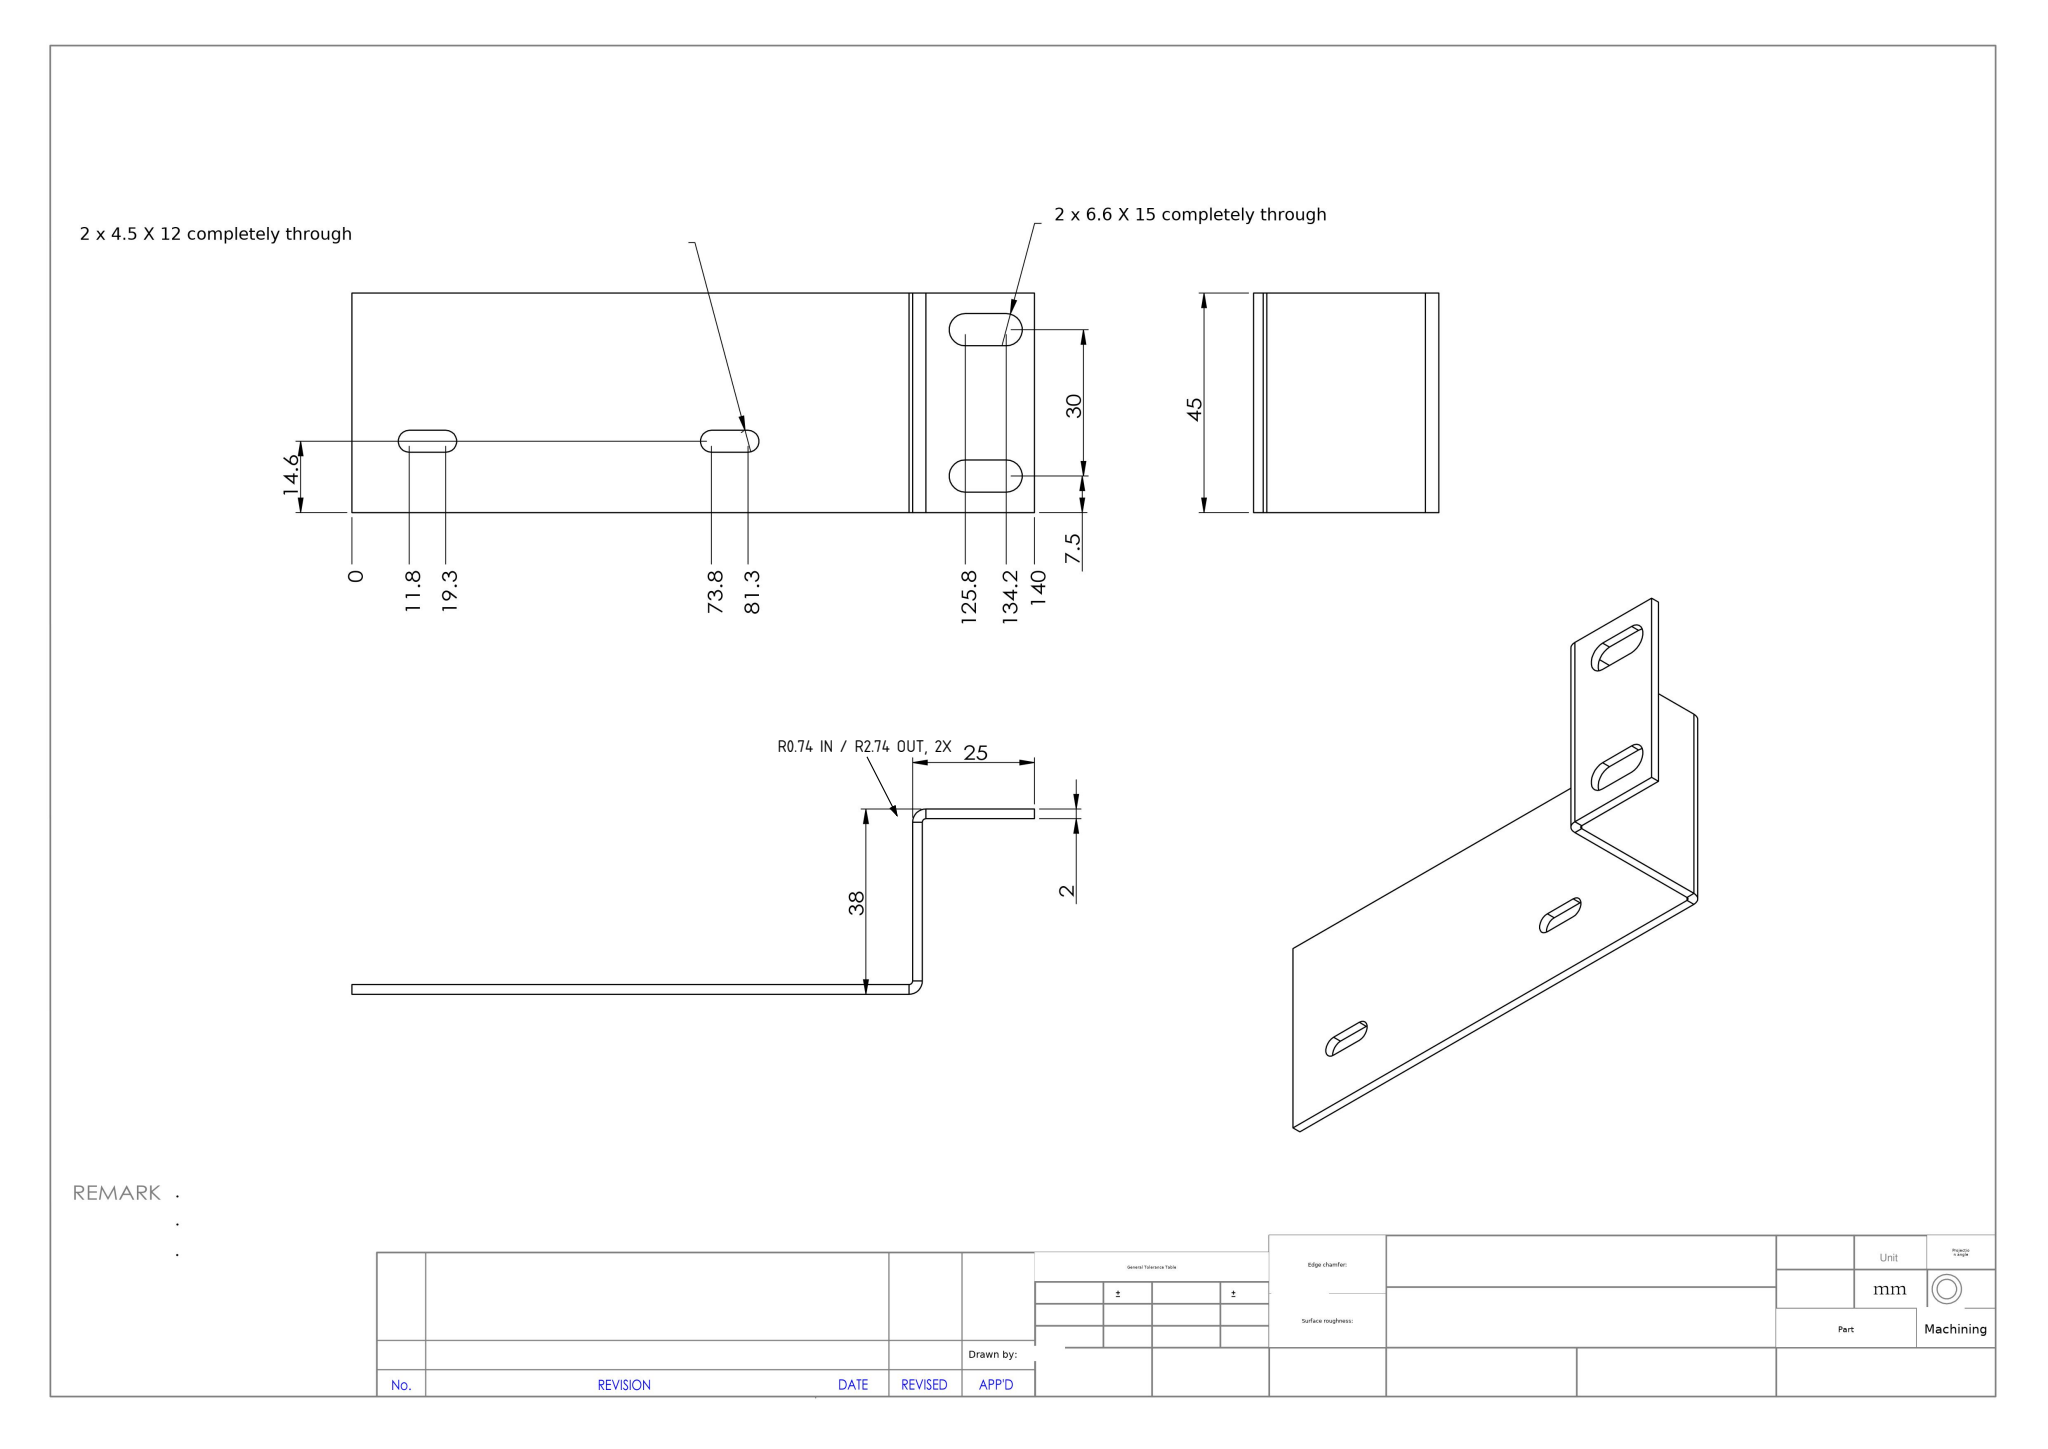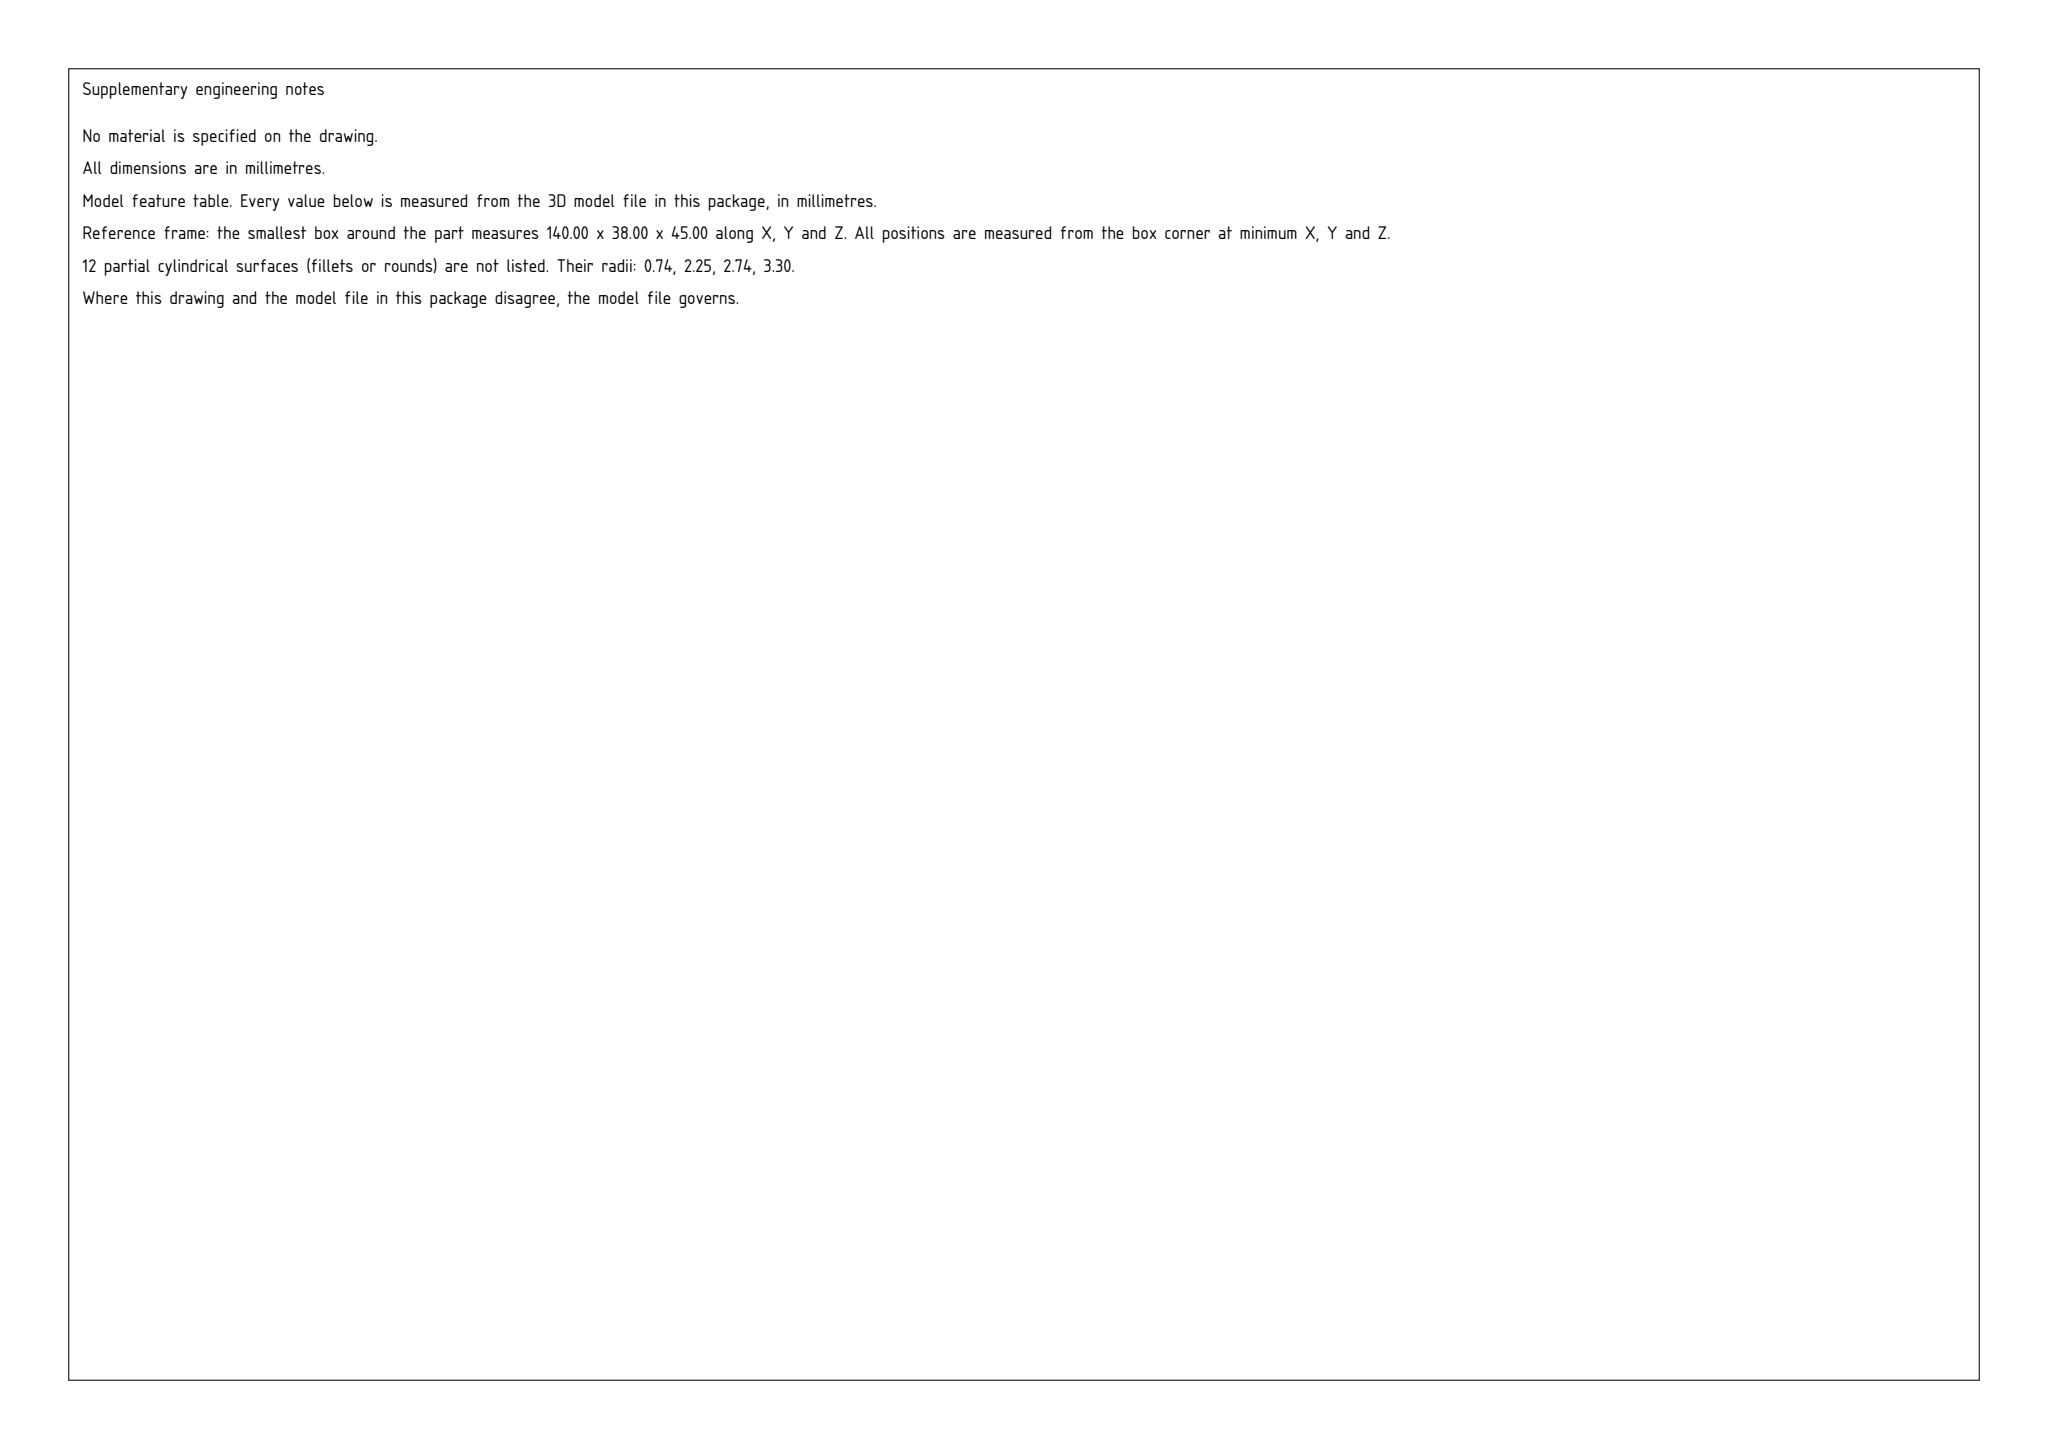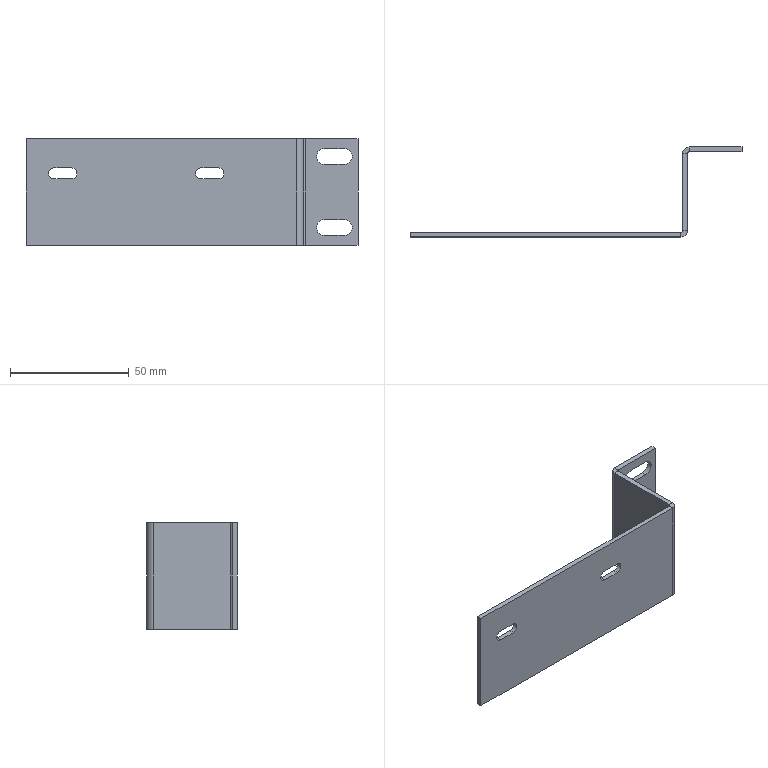Part | SolidWorks | mm | 1 solid | 38 faces | box 140 x 38 x 45 mm | volume 15149 mm3 | plane 26 | cylinder 12 | commonest cylinder face diameters 6.6 x4 4.5 x4 5.473 x2 1.473 x2
Drawing notes:
BENDS: R0.74 INSIDE, R2.74 OUTSIDE, 2 PLCS (T2) | from the solid: Cylinders dia 1.473 (R0.74) and dia 5.473 (R2.74), axis z, at (114.26,2.74) and (117.74,35.26), len 45; wall planes y=0/2 and 36/38, x=115/117